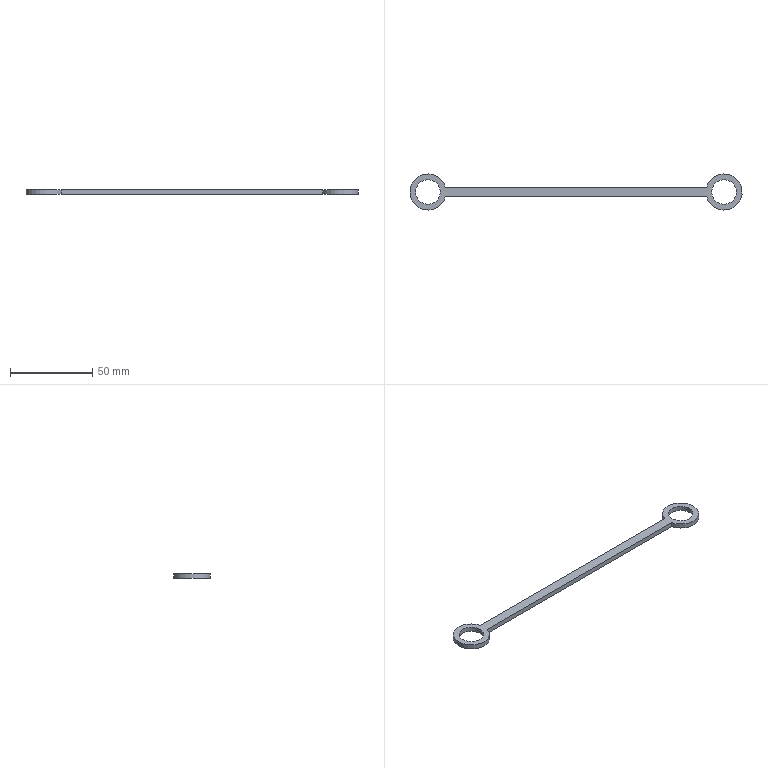Component | NX | CON_ROD3_2 | 1 solid | 8 faces | box 202 x 22 x 3 mm | volume 4069 mm3 | cylinder 4 | plane 4 | commonest cylinder face diameters 22 x2 15 x2
STEP:
#1=CARTESIAN_POINT('',(0.,0.,0.));
#2=DIRECTION('',(0.,0.,1.));
#3=DIRECTION('',(1.,0.,0.));
#4=AXIS2_PLACEMENT_3D('',#1,#2,#3);
#5=CARTESIAN_POINT('',(7.583,3.,10.));
#6=VERTEX_POINT('',#5);
#7=CARTESIAN_POINT('',(7.583,-3.,10.));
#8=VERTEX_POINT('',#7);
#9=CARTESIAN_POINT('',(-3.,-0.,10.));
#10=DIRECTION('',(0.,0.,1.));
#11=DIRECTION('',(1.,0.,0.));
#12=AXIS2_PLACEMENT_3D('',#9,#10,#11);
#13=CIRCLE('',#12,11.);
#14=CARTESIAN_POINT('',(-3.,-0.,13.));
#15=DIRECTION('',(0.,0.,-1.));
#16=DIRECTION('',(-1.,0.,0.));
#17=AXIS2_PLACEMENT_3D('',#14,#15,#16);
#18=CYLINDRICAL_SURFACE('',#17,11.);
#19=CARTESIAN_POINT('',(3.142,3.));
#20=DIRECTION('',(-1.,0.));
#21=VECTOR('',#20,1.);
#22=LINE('',#19,#21);
#23=(GEOMETRIC_REPRESENTATION_CONTEXT(2)PARAMETRIC_REPRESENTATION_CONTEXT()REPRESENTATION_CONTEXT('',''));
#24=DEFINITIONAL_REPRESENTATION('',(#22),#23);
#25=PCURVE('',#18,#24);
#26=CARTESIAN_POINT('',(-3.,-0.,10.));
#27=DIRECTION('',(0.,0.,1.));
#28=DIRECTION('',(1.,0.,0.));
#29=AXIS2_PLACEMENT_3D('',#26,#27,#28);
#30=PLANE('',#29);
#31=CARTESIAN_POINT('',(0.,0.));
#32=DIRECTION('',(1.,0.));
#33=AXIS2_PLACEMENT_2D('',#31,#32);
#34=CIRCLE('',#33,11.);
#35=(GEOMETRIC_REPRESENTATION_CONTEXT(2)PARAMETRIC_REPRESENTATION_CONTEXT()REPRESENTATION_CONTEXT('',''));
#36=DEFINITIONAL_REPRESENTATION('',(#34),#35);
#37=PCURVE('',#30,#36);
#38=SURFACE_CURVE('',#13,(#25,#37),.PCURVE_S1.);
#39=EDGE_CURVE('',#6,#8,#38,.T.);
#40=ORIENTED_EDGE('',*,*,#39,.T.);
#41=CARTESIAN_POINT('',(7.583,-3.,13.));
#42=VERTEX_POINT('',#41);
#43=CARTESIAN_POINT('',(7.583,-3.,13.));
#44=DIRECTION('',(0.,0.,-1.));
#45=VECTOR('',#44,1.);
#46=LINE('',#43,#45);
#47=CARTESIAN_POINT('',(-2.865,0.));
#48=DIRECTION('',(0.,1.));
#49=VECTOR('',#48,1.);
#50=LINE('',#47,#49);
#51=(GEOMETRIC_REPRESENTATION_CONTEXT(2)PARAMETRIC_REPRESENTATION_CONTEXT()REPRESENTATION_CONTEXT('',''));
#52=DEFINITIONAL_REPRESENTATION('',(#50),#51);
#53=PCURVE('',#18,#52);
#54=CARTESIAN_POINT('',(7.583,-3.,13.));
#55=DIRECTION('',(0.,1.,0.));
#56=DIRECTION('',(0.,0.,1.));
#57=AXIS2_PLACEMENT_3D('',#54,#55,#56);
#58=PLANE('',#57);
#59=CARTESIAN_POINT('',(0.,-0.));
#60=DIRECTION('',(-1.,0.));
#61=VECTOR('',#60,1.);
#62=LINE('',#59,#61);
#63=(GEOMETRIC_REPRESENTATION_CONTEXT(2)PARAMETRIC_REPRESENTATION_CONTEXT()REPRESENTATION_CONTEXT('',''));
#64=DEFINITIONAL_REPRESENTATION('',(#62),#63);
#65=PCURVE('',#58,#64);
#66=SURFACE_CURVE('',#46,(#53,#65),.PCURVE_S1.);
#67=EDGE_CURVE('',#42,#8,#66,.T.);
#68=ORIENTED_EDGE('',*,*,#67,.F.);
#69=CARTESIAN_POINT('',(7.583,3.,13.));
#70=VERTEX_POINT('',#69);
#71=CARTESIAN_POINT('',(-3.,-0.,13.));
#72=DIRECTION('',(0.,0.,1.));
#73=DIRECTION('',(1.,0.,0.));
#74=AXIS2_PLACEMENT_3D('',#71,#72,#73);
#75=CIRCLE('',#74,11.);
#76=CARTESIAN_POINT('',(3.142,0.));
#77=DIRECTION('',(-1.,0.));
#78=VECTOR('',#77,1.);
#79=LINE('',#76,#78);
#80=(GEOMETRIC_REPRESENTATION_CONTEXT(2)PARAMETRIC_REPRESENTATION_CONTEXT()REPRESENTATION_CONTEXT('',''));
#81=DEFINITIONAL_REPRESENTATION('',(#79),#80);
#82=PCURVE('',#18,#81);
#83=CARTESIAN_POINT('',(-3.,-0.,13.));
#84=DIRECTION('',(0.,0.,1.));
#85=DIRECTION('',(1.,0.,0.));
#86=AXIS2_PLACEMENT_3D('',#83,#84,#85);
#87=PLANE('',#86);
#88=CARTESIAN_POINT('',(0.,0.));
#89=DIRECTION('',(1.,0.));
#90=AXIS2_PLACEMENT_2D('',#88,#89);
#91=CIRCLE('',#90,11.);
#92=(GEOMETRIC_REPRESENTATION_CONTEXT(2)PARAMETRIC_REPRESENTATION_CONTEXT()REPRESENTATION_CONTEXT('',''));
#93=DEFINITIONAL_REPRESENTATION('',(#91),#92);
#94=PCURVE('',#87,#93);
#95=SURFACE_CURVE('',#75,(#82,#94),.PCURVE_S1.);
#96=EDGE_CURVE('',#70,#42,#95,.T.);
#97=ORIENTED_EDGE('',*,*,#96,.F.);
#98=CARTESIAN_POINT('',(7.583,3.,13.));
#99=DIRECTION('',(0.,0.,-1.));
#100=VECTOR('',#99,1.);
#101=LINE('',#98,#100);
#102=CARTESIAN_POINT('',(2.865,0.));
#103=DIRECTION('',(0.,1.));
#104=VECTOR('',#103,1.);
#105=LINE('',#102,#104);
#106=(GEOMETRIC_REPRESENTATION_CONTEXT(2)PARAMETRIC_REPRESENTATION_CONTEXT()REPRESENTATION_CONTEXT('',''));
#107=DEFINITIONAL_REPRESENTATION('',(#105),#106);
#108=PCURVE('',#18,#107);
#109=CARTESIAN_POINT('',(166.417,3.,13.));
#110=DIRECTION('',(0.,-1.,0.));
#111=DIRECTION('',(0.,0.,-1.));
#112=AXIS2_PLACEMENT_3D('',#109,#110,#111);
#113=PLANE('',#112);
#114=CARTESIAN_POINT('',(0.,-158.834));
#115=DIRECTION('',(1.,0.));
#116=VECTOR('',#115,1.);
#117=LINE('',#114,#116);
#118=(GEOMETRIC_REPRESENTATION_CONTEXT(2)PARAMETRIC_REPRESENTATION_CONTEXT()REPRESENTATION_CONTEXT('',''));
#119=DEFINITIONAL_REPRESENTATION('',(#117),#118);
#120=PCURVE('',#113,#119);
#121=SURFACE_CURVE('',#101,(#108,#120),.PCURVE_S1.);
#122=EDGE_CURVE('',#70,#6,#121,.T.);
#123=ORIENTED_EDGE('',*,*,#122,.T.);
#124=EDGE_LOOP('',(#40,#68,#97,#123));
#125=FACE_BOUND('',#124,.T.);
#126=ADVANCED_FACE('',(#125),#18,.T.);
#127=CARTESIAN_POINT('',(166.417,-3.,10.));
#128=VERTEX_POINT('',#127);
#129=CARTESIAN_POINT('',(7.583,-3.,10.));
#130=DIRECTION('',(1.,0.,0.));
#131=VECTOR('',#130,1.);
#132=LINE('',#129,#131);
#133=CARTESIAN_POINT('',(-3.,0.));
#134=DIRECTION('',(0.,1.));
#135=VECTOR('',#134,1.);
#136=LINE('',#133,#135);
#137=(GEOMETRIC_REPRESENTATION_CONTEXT(2)PARAMETRIC_REPRESENTATION_CONTEXT()REPRESENTATION_CONTEXT('',''));
#138=DEFINITIONAL_REPRESENTATION('',(#136),#137);
#139=PCURVE('',#58,#138);
#140=CARTESIAN_POINT('',(10.583,-3.));
#141=DIRECTION('',(1.,0.));
#142=VECTOR('',#141,1.);
#143=LINE('',#140,#142);
#144=(GEOMETRIC_REPRESENTATION_CONTEXT(2)PARAMETRIC_REPRESENTATION_CONTEXT()REPRESENTATION_CONTEXT('',''));
#145=DEFINITIONAL_REPRESENTATION('',(#143),#144);
#146=PCURVE('',#30,#145);
#147=SURFACE_CURVE('',#132,(#139,#146),.PCURVE_S1.);
#148=EDGE_CURVE('',#8,#128,#147,.T.);
#149=ORIENTED_EDGE('',*,*,#148,.T.);
#150=CARTESIAN_POINT('',(166.417,-3.,13.));
#151=VERTEX_POINT('',#150);
#152=CARTESIAN_POINT('',(166.417,-3.,13.));
#153=DIRECTION('',(0.,0.,-1.));
#154=VECTOR('',#153,1.);
#155=LINE('',#152,#154);
#156=CARTESIAN_POINT('',(0.,158.834));
#157=DIRECTION('',(-1.,0.));
#158=VECTOR('',#157,1.);
#159=LINE('',#156,#158);
#160=(GEOMETRIC_REPRESENTATION_CONTEXT(2)PARAMETRIC_REPRESENTATION_CONTEXT()REPRESENTATION_CONTEXT('',''));
#161=DEFINITIONAL_REPRESENTATION('',(#159),#160);
#162=PCURVE('',#58,#161);
#163=CARTESIAN_POINT('',(177.,-0.,13.));
#164=DIRECTION('',(0.,0.,-1.));
#165=DIRECTION('',(-1.,0.,0.));
#166=AXIS2_PLACEMENT_3D('',#163,#164,#165);
#167=CYLINDRICAL_SURFACE('',#166,11.);
#168=CARTESIAN_POINT('',(6.007,0.));
#169=DIRECTION('',(0.,1.));
#170=VECTOR('',#169,1.);
#171=LINE('',#168,#170);
#172=(GEOMETRIC_REPRESENTATION_CONTEXT(2)PARAMETRIC_REPRESENTATION_CONTEXT()REPRESENTATION_CONTEXT('',''));
#173=DEFINITIONAL_REPRESENTATION('',(#171),#172);
#174=PCURVE('',#167,#173);
#175=SURFACE_CURVE('',#155,(#162,#174),.PCURVE_S1.);
#176=EDGE_CURVE('',#151,#128,#175,.T.);
#177=ORIENTED_EDGE('',*,*,#176,.F.);
#178=CARTESIAN_POINT('',(7.583,-3.,13.));
#179=DIRECTION('',(1.,0.,0.));
#180=VECTOR('',#179,1.);
#181=LINE('',#178,#180);
#182=CARTESIAN_POINT('',(0.,0.));
#183=DIRECTION('',(0.,1.));
#184=VECTOR('',#183,1.);
#185=LINE('',#182,#184);
#186=(GEOMETRIC_REPRESENTATION_CONTEXT(2)PARAMETRIC_REPRESENTATION_CONTEXT()REPRESENTATION_CONTEXT('',''));
#187=DEFINITIONAL_REPRESENTATION('',(#185),#186);
#188=PCURVE('',#58,#187);
#189=CARTESIAN_POINT('',(10.583,-3.));
#190=DIRECTION('',(1.,0.));
#191=VECTOR('',#190,1.);
#192=LINE('',#189,#191);
#193=(GEOMETRIC_REPRESENTATION_CONTEXT(2)PARAMETRIC_REPRESENTATION_CONTEXT()REPRESENTATION_CONTEXT('',''));
#194=DEFINITIONAL_REPRESENTATION('',(#192),#193);
#195=PCURVE('',#87,#194);
#196=SURFACE_CURVE('',#181,(#188,#195),.PCURVE_S1.);
#197=EDGE_CURVE('',#42,#151,#196,.T.);
#198=ORIENTED_EDGE('',*,*,#197,.F.);
#199=ORIENTED_EDGE('',*,*,#67,.T.);
#200=EDGE_LOOP('',(#149,#177,#198,#199));
#201=FACE_BOUND('',#200,.T.);
#202=ADVANCED_FACE('',(#201),#58,.F.);
#203=CARTESIAN_POINT('',(166.417,3.,10.));
#204=VERTEX_POINT('',#203);
#205=CARTESIAN_POINT('',(177.,-0.,10.));
#206=DIRECTION('',(0.,0.,1.));
#207=DIRECTION('',(1.,0.,0.));
#208=AXIS2_PLACEMENT_3D('',#205,#206,#207);
#209=CIRCLE('',#208,11.);
#210=CARTESIAN_POINT('',(9.425,3.));
#211=DIRECTION('',(-1.,0.));
#212=VECTOR('',#211,1.);
#213=LINE('',#210,#212);
#214=(GEOMETRIC_REPRESENTATION_CONTEXT(2)PARAMETRIC_REPRESENTATION_CONTEXT()REPRESENTATION_CONTEXT('',''));
#215=DEFINITIONAL_REPRESENTATION('',(#213),#214);
#216=PCURVE('',#167,#215);
#217=CARTESIAN_POINT('',(180.,0.));
#218=DIRECTION('',(1.,0.));
#219=AXIS2_PLACEMENT_2D('',#217,#218);
#220=CIRCLE('',#219,11.);
#221=(GEOMETRIC_REPRESENTATION_CONTEXT(2)PARAMETRIC_REPRESENTATION_CONTEXT()REPRESENTATION_CONTEXT('',''));
#222=DEFINITIONAL_REPRESENTATION('',(#220),#221);
#223=PCURVE('',#30,#222);
#224=SURFACE_CURVE('',#209,(#216,#223),.PCURVE_S1.);
#225=EDGE_CURVE('',#128,#204,#224,.T.);
#226=ORIENTED_EDGE('',*,*,#225,.T.);
#227=CARTESIAN_POINT('',(166.417,3.,13.));
#228=VERTEX_POINT('',#227);
#229=CARTESIAN_POINT('',(166.417,3.,13.));
#230=DIRECTION('',(0.,0.,-1.));
#231=VECTOR('',#230,1.);
#232=LINE('',#229,#231);
#233=CARTESIAN_POINT('',(0.2762,0.));
#234=DIRECTION('',(0.,1.));
#235=VECTOR('',#234,1.);
#236=LINE('',#233,#235);
#237=(GEOMETRIC_REPRESENTATION_CONTEXT(2)PARAMETRIC_REPRESENTATION_CONTEXT()REPRESENTATION_CONTEXT('',''));
#238=DEFINITIONAL_REPRESENTATION('',(#236),#237);
#239=PCURVE('',#167,#238);
#240=CARTESIAN_POINT('',(0.,-0.));
#241=DIRECTION('',(1.,0.));
#242=VECTOR('',#241,1.);
#243=LINE('',#240,#242);
#244=(GEOMETRIC_REPRESENTATION_CONTEXT(2)PARAMETRIC_REPRESENTATION_CONTEXT()REPRESENTATION_CONTEXT('',''));
#245=DEFINITIONAL_REPRESENTATION('',(#243),#244);
#246=PCURVE('',#113,#245);
#247=SURFACE_CURVE('',#232,(#239,#246),.PCURVE_S1.);
#248=EDGE_CURVE('',#228,#204,#247,.T.);
#249=ORIENTED_EDGE('',*,*,#248,.F.);
#250=CARTESIAN_POINT('',(177.,-0.,13.));
#251=DIRECTION('',(0.,0.,1.));
#252=DIRECTION('',(1.,0.,0.));
#253=AXIS2_PLACEMENT_3D('',#250,#251,#252);
#254=CIRCLE('',#253,11.);
#255=CARTESIAN_POINT('',(9.425,0.));
#256=DIRECTION('',(-1.,0.));
#257=VECTOR('',#256,1.);
#258=LINE('',#255,#257);
#259=(GEOMETRIC_REPRESENTATION_CONTEXT(2)PARAMETRIC_REPRESENTATION_CONTEXT()REPRESENTATION_CONTEXT('',''));
#260=DEFINITIONAL_REPRESENTATION('',(#258),#259);
#261=PCURVE('',#167,#260);
#262=CARTESIAN_POINT('',(180.,0.));
#263=DIRECTION('',(1.,0.));
#264=AXIS2_PLACEMENT_2D('',#262,#263);
#265=CIRCLE('',#264,11.);
#266=(GEOMETRIC_REPRESENTATION_CONTEXT(2)PARAMETRIC_REPRESENTATION_CONTEXT()REPRESENTATION_CONTEXT('',''));
#267=DEFINITIONAL_REPRESENTATION('',(#265),#266);
#268=PCURVE('',#87,#267);
#269=SURFACE_CURVE('',#254,(#261,#268),.PCURVE_S1.);
#270=EDGE_CURVE('',#151,#228,#269,.T.);
#271=ORIENTED_EDGE('',*,*,#270,.F.);
#272=ORIENTED_EDGE('',*,*,#176,.T.);
#273=EDGE_LOOP('',(#226,#249,#271,#272));
#274=FACE_BOUND('',#273,.T.);
#275=ADVANCED_FACE('',(#274),#167,.T.);
#276=CARTESIAN_POINT('',(4.5,-0.,13.));
#277=VERTEX_POINT('',#276);
#278=CARTESIAN_POINT('',(-3.,-0.,13.));
#279=DIRECTION('',(0.,0.,1.));
#280=DIRECTION('',(1.,0.,0.));
#281=AXIS2_PLACEMENT_3D('',#278,#279,#280);
#282=CIRCLE('',#281,7.5);
#283=CARTESIAN_POINT('',(-3.,-0.,13.));
#284=DIRECTION('',(0.,0.,-1.));
#285=DIRECTION('',(-1.,0.,0.));
#286=AXIS2_PLACEMENT_3D('',#283,#284,#285);
#287=CYLINDRICAL_SURFACE('',#286,7.5);
#288=CARTESIAN_POINT('',(9.425,0.));
#289=DIRECTION('',(-1.,0.));
#290=VECTOR('',#289,1.);
#291=LINE('',#288,#290);
#292=(GEOMETRIC_REPRESENTATION_CONTEXT(2)PARAMETRIC_REPRESENTATION_CONTEXT()REPRESENTATION_CONTEXT('',''));
#293=DEFINITIONAL_REPRESENTATION('',(#291),#292);
#294=PCURVE('',#287,#293);
#295=CARTESIAN_POINT('',(0.,0.));
#296=DIRECTION('',(1.,0.));
#297=AXIS2_PLACEMENT_2D('',#295,#296);
#298=CIRCLE('',#297,7.5);
#299=(GEOMETRIC_REPRESENTATION_CONTEXT(2)PARAMETRIC_REPRESENTATION_CONTEXT()REPRESENTATION_CONTEXT('',''));
#300=DEFINITIONAL_REPRESENTATION('',(#298),#299);
#301=PCURVE('',#87,#300);
#302=SURFACE_CURVE('',#282,(#294,#301),.PCURVE_S1.);
#303=EDGE_CURVE('',#277,#277,#302,.T.);
#304=ORIENTED_EDGE('',*,*,#303,.F.);
#305=CARTESIAN_POINT('',(4.5,-0.,10.));
#306=VERTEX_POINT('',#305);
#307=CARTESIAN_POINT('',(4.5,-0.,13.));
#308=CARTESIAN_POINT('',(4.5,-0.,10.));
#309=B_SPLINE_CURVE_WITH_KNOTS('',1,(#307,#308),.UNSPECIFIED.,.F.,.F.,(2,2),(0.,3.),.PIECEWISE_BEZIER_KNOTS.);
#310=CARTESIAN_POINT('',(9.425,0.));
#311=DIRECTION('',(0.,1.));
#312=VECTOR('',#311,1.);
#313=LINE('',#310,#312);
#314=(GEOMETRIC_REPRESENTATION_CONTEXT(2)PARAMETRIC_REPRESENTATION_CONTEXT()REPRESENTATION_CONTEXT('',''));
#315=DEFINITIONAL_REPRESENTATION('',(#313),#314);
#316=PCURVE('',#287,#315);
#317=CARTESIAN_POINT('',(3.142,0.));
#318=DIRECTION('',(0.,1.));
#319=VECTOR('',#318,1.);
#320=LINE('',#317,#319);
#321=(GEOMETRIC_REPRESENTATION_CONTEXT(2)PARAMETRIC_REPRESENTATION_CONTEXT()REPRESENTATION_CONTEXT('',''));
#322=DEFINITIONAL_REPRESENTATION('',(#320),#321);
#323=PCURVE('',#287,#322);
#324=SEAM_CURVE('',#309,(#316,#323),.PCURVE_S1.);
#325=EDGE_CURVE('',#277,#306,#324,.T.);
#326=ORIENTED_EDGE('',*,*,#325,.T.);
#327=CARTESIAN_POINT('',(-3.,-0.,10.));
#328=DIRECTION('',(0.,0.,1.));
#329=DIRECTION('',(1.,0.,0.));
#330=AXIS2_PLACEMENT_3D('',#327,#328,#329);
#331=CIRCLE('',#330,7.5);
#332=CARTESIAN_POINT('',(9.425,3.));
#333=DIRECTION('',(-1.,0.));
#334=VECTOR('',#333,1.);
#335=LINE('',#332,#334);
#336=(GEOMETRIC_REPRESENTATION_CONTEXT(2)PARAMETRIC_REPRESENTATION_CONTEXT()REPRESENTATION_CONTEXT('',''));
#337=DEFINITIONAL_REPRESENTATION('',(#335),#336);
#338=PCURVE('',#287,#337);
#339=CARTESIAN_POINT('',(0.,0.));
#340=DIRECTION('',(1.,0.));
#341=AXIS2_PLACEMENT_2D('',#339,#340);
#342=CIRCLE('',#341,7.5);
#343=(GEOMETRIC_REPRESENTATION_CONTEXT(2)PARAMETRIC_REPRESENTATION_CONTEXT()REPRESENTATION_CONTEXT('',''));
#344=DEFINITIONAL_REPRESENTATION('',(#342),#343);
#345=PCURVE('',#30,#344);
#346=SURFACE_CURVE('',#331,(#338,#345),.PCURVE_S1.);
#347=EDGE_CURVE('',#306,#306,#346,.T.);
#348=ORIENTED_EDGE('',*,*,#347,.T.);
#349=ORIENTED_EDGE('',*,*,#325,.F.);
#350=EDGE_LOOP('',(#304,#326,#348,#349));
#351=FACE_BOUND('',#350,.F.);
#352=ADVANCED_FACE('',(#351),#287,.F.);
#353=CARTESIAN_POINT('',(166.417,3.,10.));
#354=DIRECTION('',(-1.,0.,0.));
#355=VECTOR('',#354,1.);
#356=LINE('',#353,#355);
#357=CARTESIAN_POINT('',(3.,0.));
#358=DIRECTION('',(0.,-1.));
#359=VECTOR('',#358,1.);
#360=LINE('',#357,#359);
#361=(GEOMETRIC_REPRESENTATION_CONTEXT(2)PARAMETRIC_REPRESENTATION_CONTEXT()REPRESENTATION_CONTEXT('',''));
#362=DEFINITIONAL_REPRESENTATION('',(#360),#361);
#363=PCURVE('',#113,#362);
#364=CARTESIAN_POINT('',(169.417,3.));
#365=DIRECTION('',(-1.,0.));
#366=VECTOR('',#365,1.);
#367=LINE('',#364,#366);
#368=(GEOMETRIC_REPRESENTATION_CONTEXT(2)PARAMETRIC_REPRESENTATION_CONTEXT()REPRESENTATION_CONTEXT('',''));
#369=DEFINITIONAL_REPRESENTATION('',(#367),#368);
#370=PCURVE('',#30,#369);
#371=SURFACE_CURVE('',#356,(#363,#370),.PCURVE_S1.);
#372=EDGE_CURVE('',#204,#6,#371,.T.);
#373=ORIENTED_EDGE('',*,*,#372,.T.);
#374=ORIENTED_EDGE('',*,*,#122,.F.);
#375=CARTESIAN_POINT('',(166.417,3.,13.));
#376=DIRECTION('',(-1.,0.,0.));
#377=VECTOR('',#376,1.);
#378=LINE('',#375,#377);
#379=CARTESIAN_POINT('',(0.,0.));
#380=DIRECTION('',(0.,-1.));
#381=VECTOR('',#380,1.);
#382=LINE('',#379,#381);
#383=(GEOMETRIC_REPRESENTATION_CONTEXT(2)PARAMETRIC_REPRESENTATION_CONTEXT()REPRESENTATION_CONTEXT('',''));
#384=DEFINITIONAL_REPRESENTATION('',(#382),#383);
#385=PCURVE('',#113,#384);
#386=CARTESIAN_POINT('',(169.417,3.));
#387=DIRECTION('',(-1.,0.));
#388=VECTOR('',#387,1.);
#389=LINE('',#386,#388);
#390=(GEOMETRIC_REPRESENTATION_CONTEXT(2)PARAMETRIC_REPRESENTATION_CONTEXT()REPRESENTATION_CONTEXT('',''));
#391=DEFINITIONAL_REPRESENTATION('',(#389),#390);
#392=PCURVE('',#87,#391);
#393=SURFACE_CURVE('',#378,(#385,#392),.PCURVE_S1.);
#394=EDGE_CURVE('',#228,#70,#393,.T.);
#395=ORIENTED_EDGE('',*,*,#394,.F.);
#396=ORIENTED_EDGE('',*,*,#248,.T.);
#397=EDGE_LOOP('',(#373,#374,#395,#396));
#398=FACE_BOUND('',#397,.T.);
#399=ADVANCED_FACE('',(#398),#113,.F.);
#400=CARTESIAN_POINT('',(184.5,-0.,13.));
#401=VERTEX_POINT('',#400);
#402=CARTESIAN_POINT('',(177.,-0.,13.));
#403=DIRECTION('',(0.,0.,1.));
#404=DIRECTION('',(1.,0.,0.));
#405=AXIS2_PLACEMENT_3D('',#402,#403,#404);
#406=CIRCLE('',#405,7.5);
#407=CARTESIAN_POINT('',(177.,-0.,13.));
#408=DIRECTION('',(0.,0.,-1.));
#409=DIRECTION('',(-1.,0.,0.));
#410=AXIS2_PLACEMENT_3D('',#407,#408,#409);
#411=CYLINDRICAL_SURFACE('',#410,7.5);
#412=CARTESIAN_POINT('',(9.425,0.));
#413=DIRECTION('',(-1.,0.));
#414=VECTOR('',#413,1.);
#415=LINE('',#412,#414);
#416=(GEOMETRIC_REPRESENTATION_CONTEXT(2)PARAMETRIC_REPRESENTATION_CONTEXT()REPRESENTATION_CONTEXT('',''));
#417=DEFINITIONAL_REPRESENTATION('',(#415),#416);
#418=PCURVE('',#411,#417);
#419=CARTESIAN_POINT('',(180.,0.));
#420=DIRECTION('',(1.,0.));
#421=AXIS2_PLACEMENT_2D('',#419,#420);
#422=CIRCLE('',#421,7.5);
#423=(GEOMETRIC_REPRESENTATION_CONTEXT(2)PARAMETRIC_REPRESENTATION_CONTEXT()REPRESENTATION_CONTEXT('',''));
#424=DEFINITIONAL_REPRESENTATION('',(#422),#423);
#425=PCURVE('',#87,#424);
#426=SURFACE_CURVE('',#406,(#418,#425),.PCURVE_S1.);
#427=EDGE_CURVE('',#401,#401,#426,.T.);
#428=ORIENTED_EDGE('',*,*,#427,.F.);
#429=CARTESIAN_POINT('',(184.5,-0.,10.));
#430=VERTEX_POINT('',#429);
#431=CARTESIAN_POINT('',(184.5,-0.,13.));
#432=CARTESIAN_POINT('',(184.5,-0.,10.));
#433=B_SPLINE_CURVE_WITH_KNOTS('',1,(#431,#432),.UNSPECIFIED.,.F.,.F.,(2,2),(0.,3.),.PIECEWISE_BEZIER_KNOTS.);
#434=CARTESIAN_POINT('',(9.425,0.));
#435=DIRECTION('',(0.,1.));
#436=VECTOR('',#435,1.);
#437=LINE('',#434,#436);
#438=(GEOMETRIC_REPRESENTATION_CONTEXT(2)PARAMETRIC_REPRESENTATION_CONTEXT()REPRESENTATION_CONTEXT('',''));
#439=DEFINITIONAL_REPRESENTATION('',(#437),#438);
#440=PCURVE('',#411,#439);
#441=CARTESIAN_POINT('',(3.142,0.));
#442=DIRECTION('',(0.,1.));
#443=VECTOR('',#442,1.);
#444=LINE('',#441,#443);
#445=(GEOMETRIC_REPRESENTATION_CONTEXT(2)PARAMETRIC_REPRESENTATION_CONTEXT()REPRESENTATION_CONTEXT('',''));
#446=DEFINITIONAL_REPRESENTATION('',(#444),#445);
#447=PCURVE('',#411,#446);
#448=SEAM_CURVE('',#433,(#440,#447),.PCURVE_S1.);
#449=EDGE_CURVE('',#401,#430,#448,.T.);
#450=ORIENTED_EDGE('',*,*,#449,.T.);
#451=CARTESIAN_POINT('',(177.,-0.,10.));
#452=DIRECTION('',(0.,0.,1.));
#453=DIRECTION('',(1.,0.,0.));
#454=AXIS2_PLACEMENT_3D('',#451,#452,#453);
#455=CIRCLE('',#454,7.5);
#456=CARTESIAN_POINT('',(9.425,3.));
#457=DIRECTION('',(-1.,0.));
#458=VECTOR('',#457,1.);
#459=LINE('',#456,#458);
#460=(GEOMETRIC_REPRESENTATION_CONTEXT(2)PARAMETRIC_REPRESENTATION_CONTEXT()REPRESENTATION_CONTEXT('',''));
#461=DEFINITIONAL_REPRESENTATION('',(#459),#460);
#462=PCURVE('',#411,#461);
#463=CARTESIAN_POINT('',(180.,0.));
#464=DIRECTION('',(1.,0.));
#465=AXIS2_PLACEMENT_2D('',#463,#464);
#466=CIRCLE('',#465,7.5);
#467=(GEOMETRIC_REPRESENTATION_CONTEXT(2)PARAMETRIC_REPRESENTATION_CONTEXT()REPRESENTATION_CONTEXT('',''));
#468=DEFINITIONAL_REPRESENTATION('',(#466),#467);
#469=PCURVE('',#30,#468);
#470=SURFACE_CURVE('',#455,(#462,#469),.PCURVE_S1.);
#471=EDGE_CURVE('',#430,#430,#470,.T.);
#472=ORIENTED_EDGE('',*,*,#471,.T.);
#473=ORIENTED_EDGE('',*,*,#449,.F.);
#474=EDGE_LOOP('',(#428,#450,#472,#473));
#475=FACE_BOUND('',#474,.F.);
#476=ADVANCED_FACE('',(#475),#411,.F.);
#477=ORIENTED_EDGE('',*,*,#96,.T.);
#478=ORIENTED_EDGE('',*,*,#197,.T.);
#479=ORIENTED_EDGE('',*,*,#270,.T.);
#480=ORIENTED_EDGE('',*,*,#394,.T.);
#481=EDGE_LOOP('',(#477,#478,#479,#480));
#482=FACE_BOUND('',#481,.T.);
#483=ORIENTED_EDGE('',*,*,#303,.F.);
#484=EDGE_LOOP('',(#483));
#485=FACE_BOUND('',#484,.T.);
#486=ORIENTED_EDGE('',*,*,#427,.F.);
#487=EDGE_LOOP('',(#486));
#488=FACE_BOUND('',#487,.T.);
#489=ADVANCED_FACE('',(#482,#485,#488),#87,.T.);
#490=ORIENTED_EDGE('',*,*,#39,.F.);
#491=ORIENTED_EDGE('',*,*,#372,.F.);
#492=ORIENTED_EDGE('',*,*,#225,.F.);
#493=ORIENTED_EDGE('',*,*,#148,.F.);
#494=EDGE_LOOP('',(#490,#491,#492,#493));
#495=FACE_BOUND('',#494,.T.);
#496=ORIENTED_EDGE('',*,*,#347,.T.);
#497=EDGE_LOOP('',(#496));
#498=FACE_BOUND('',#497,.T.);
#499=ORIENTED_EDGE('',*,*,#471,.T.);
#500=EDGE_LOOP('',(#499));
#501=FACE_BOUND('',#500,.T.);
#502=ADVANCED_FACE('',(#495,#498,#501),#30,.F.);
#503=CLOSED_SHELL('',(#126,#202,#275,#352,#399,#476,#489,#502));
#504=MANIFOLD_SOLID_BREP('',#503);
#505=(LENGTH_UNIT()NAMED_UNIT(*)SI_UNIT(.MILLI.,.METRE.));
#506=UNCERTAINTY_MEASURE_WITH_UNIT(LENGTH_MEASURE(0.000002),#505,'','');
#507=(NAMED_UNIT(*)PLANE_ANGLE_UNIT()SI_UNIT($,.RADIAN.));
#508=(NAMED_UNIT(*)SI_UNIT($,.STERADIAN.)SOLID_ANGLE_UNIT());
#509=(GEOMETRIC_REPRESENTATION_CONTEXT(3)GLOBAL_UNCERTAINTY_ASSIGNED_CONTEXT((#506))GLOBAL_UNIT_ASSIGNED_CONTEXT((#505,#507,#508))REPRESENTATION_CONTEXT('',''));
#510=ADVANCED_BREP_SHAPE_REPRESENTATION('',(#4,#504),#509);